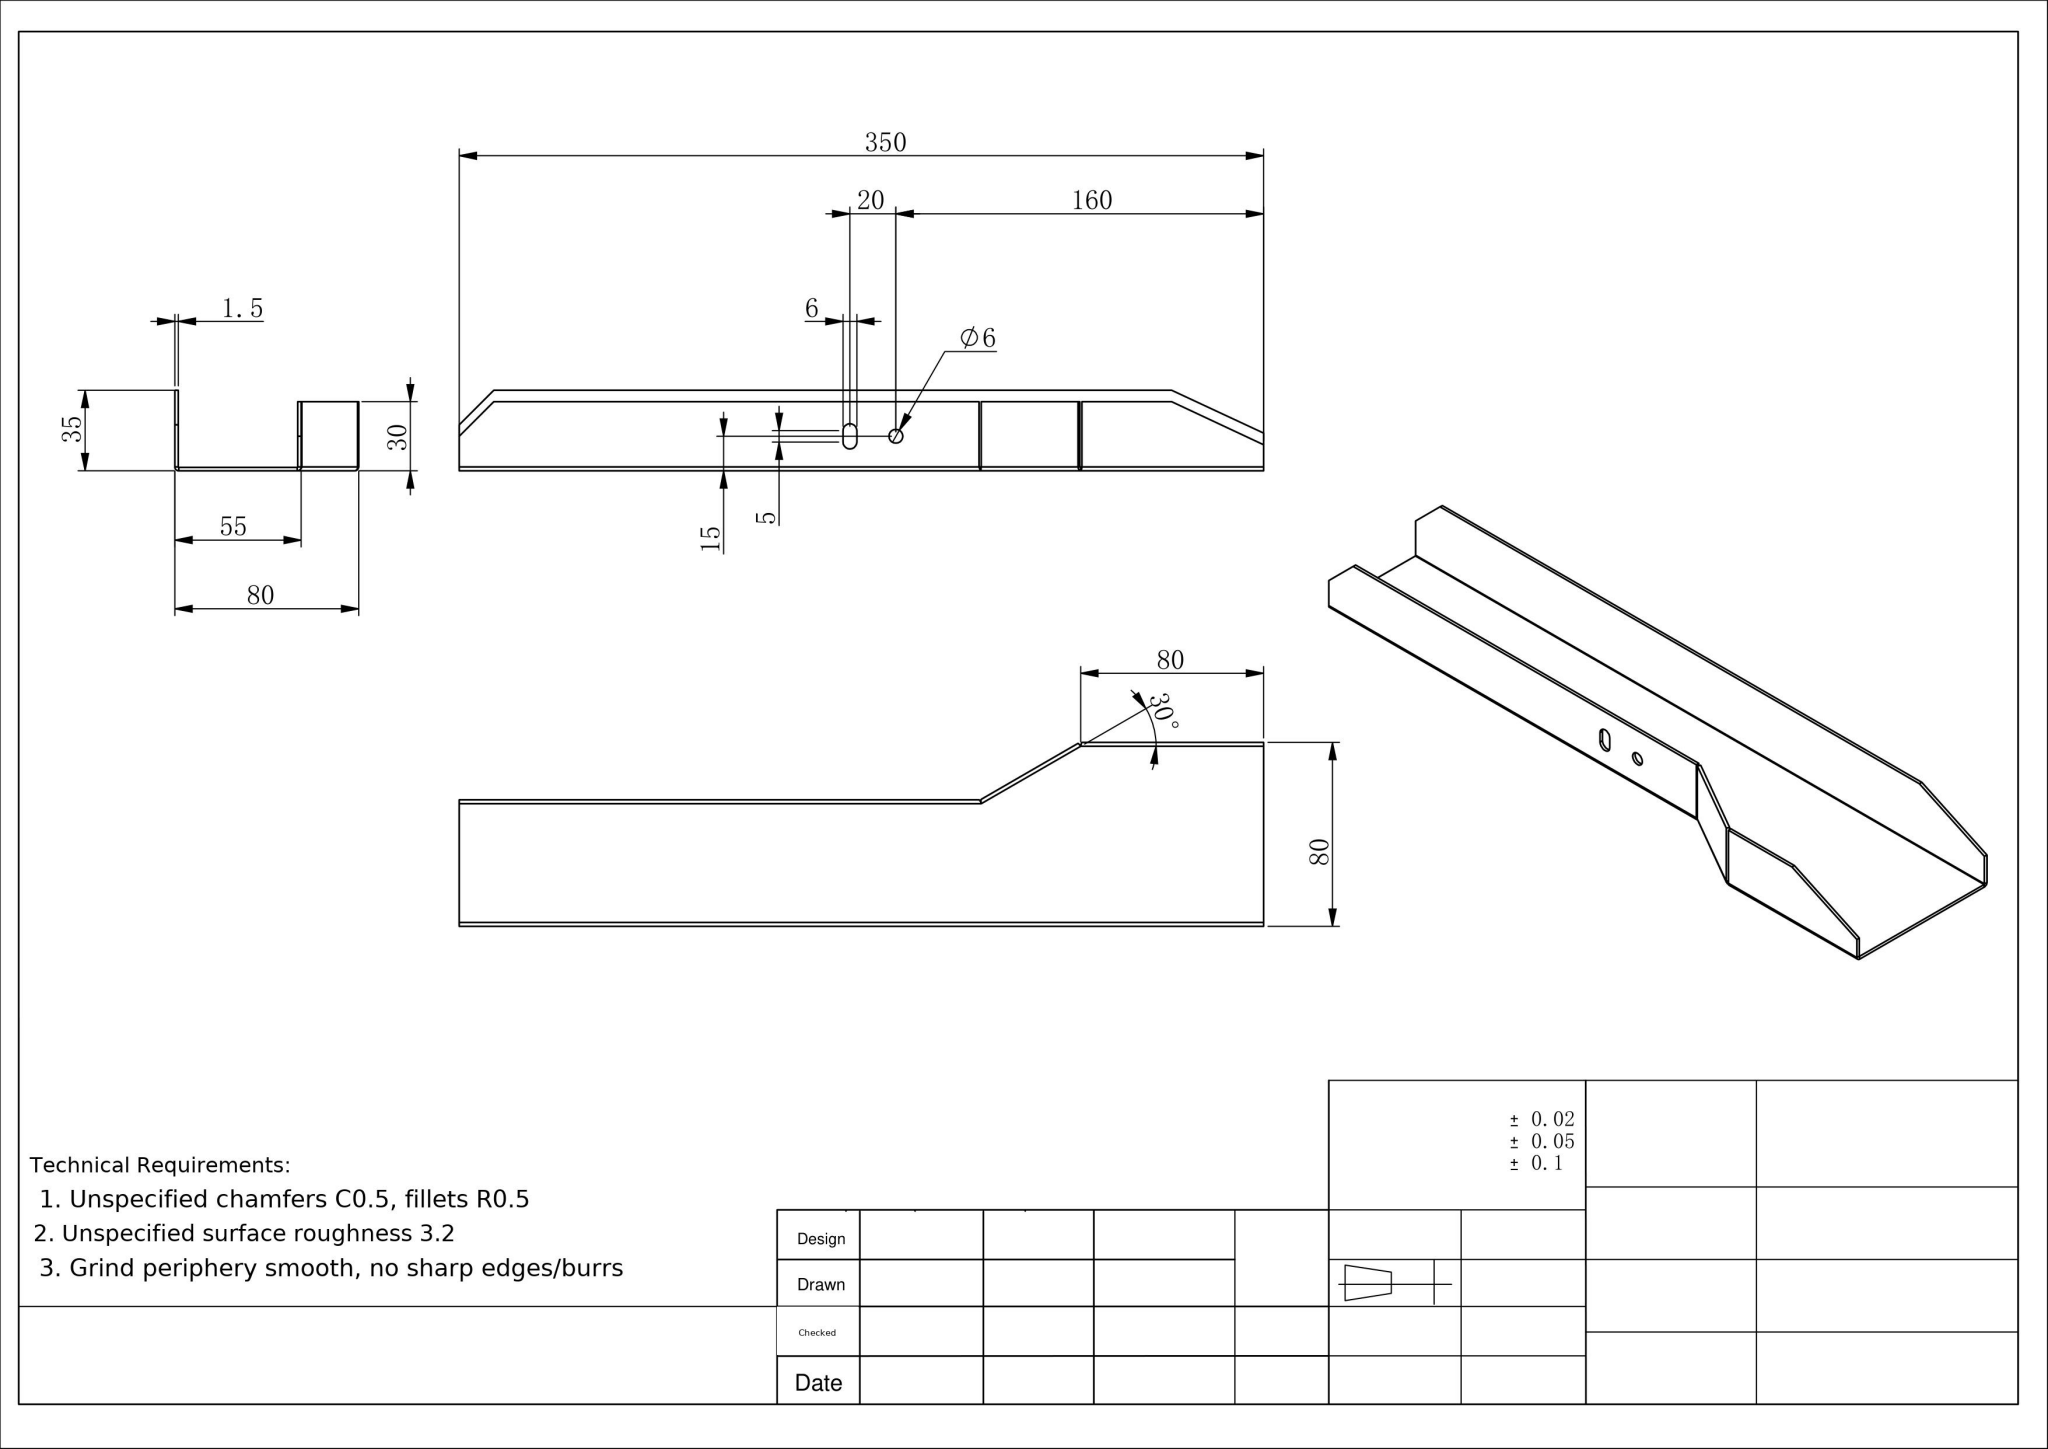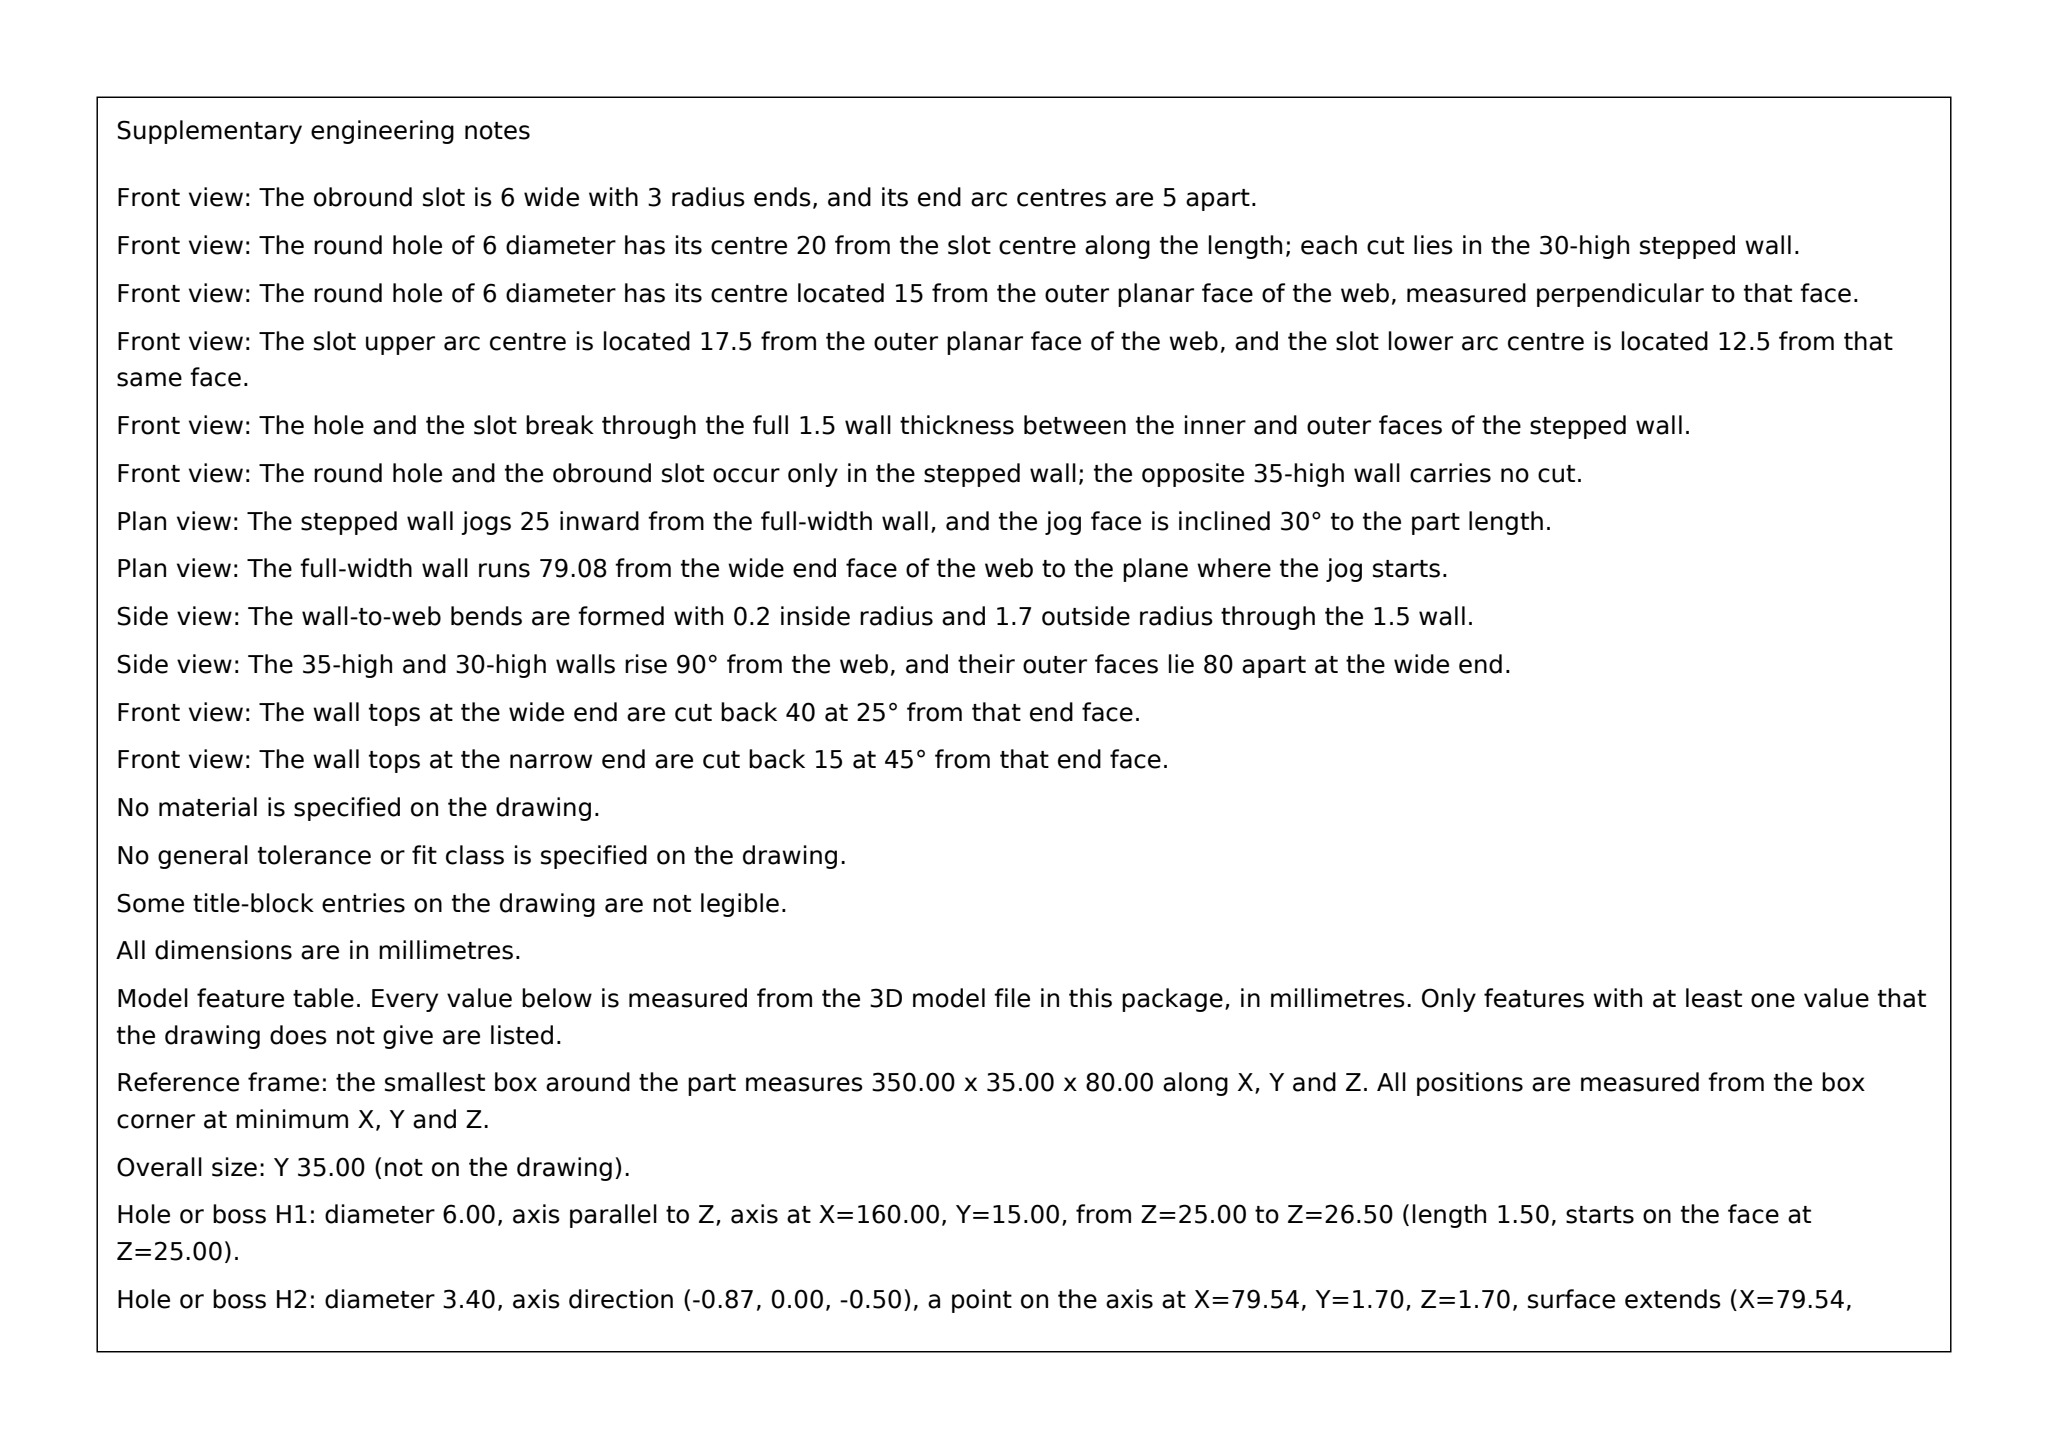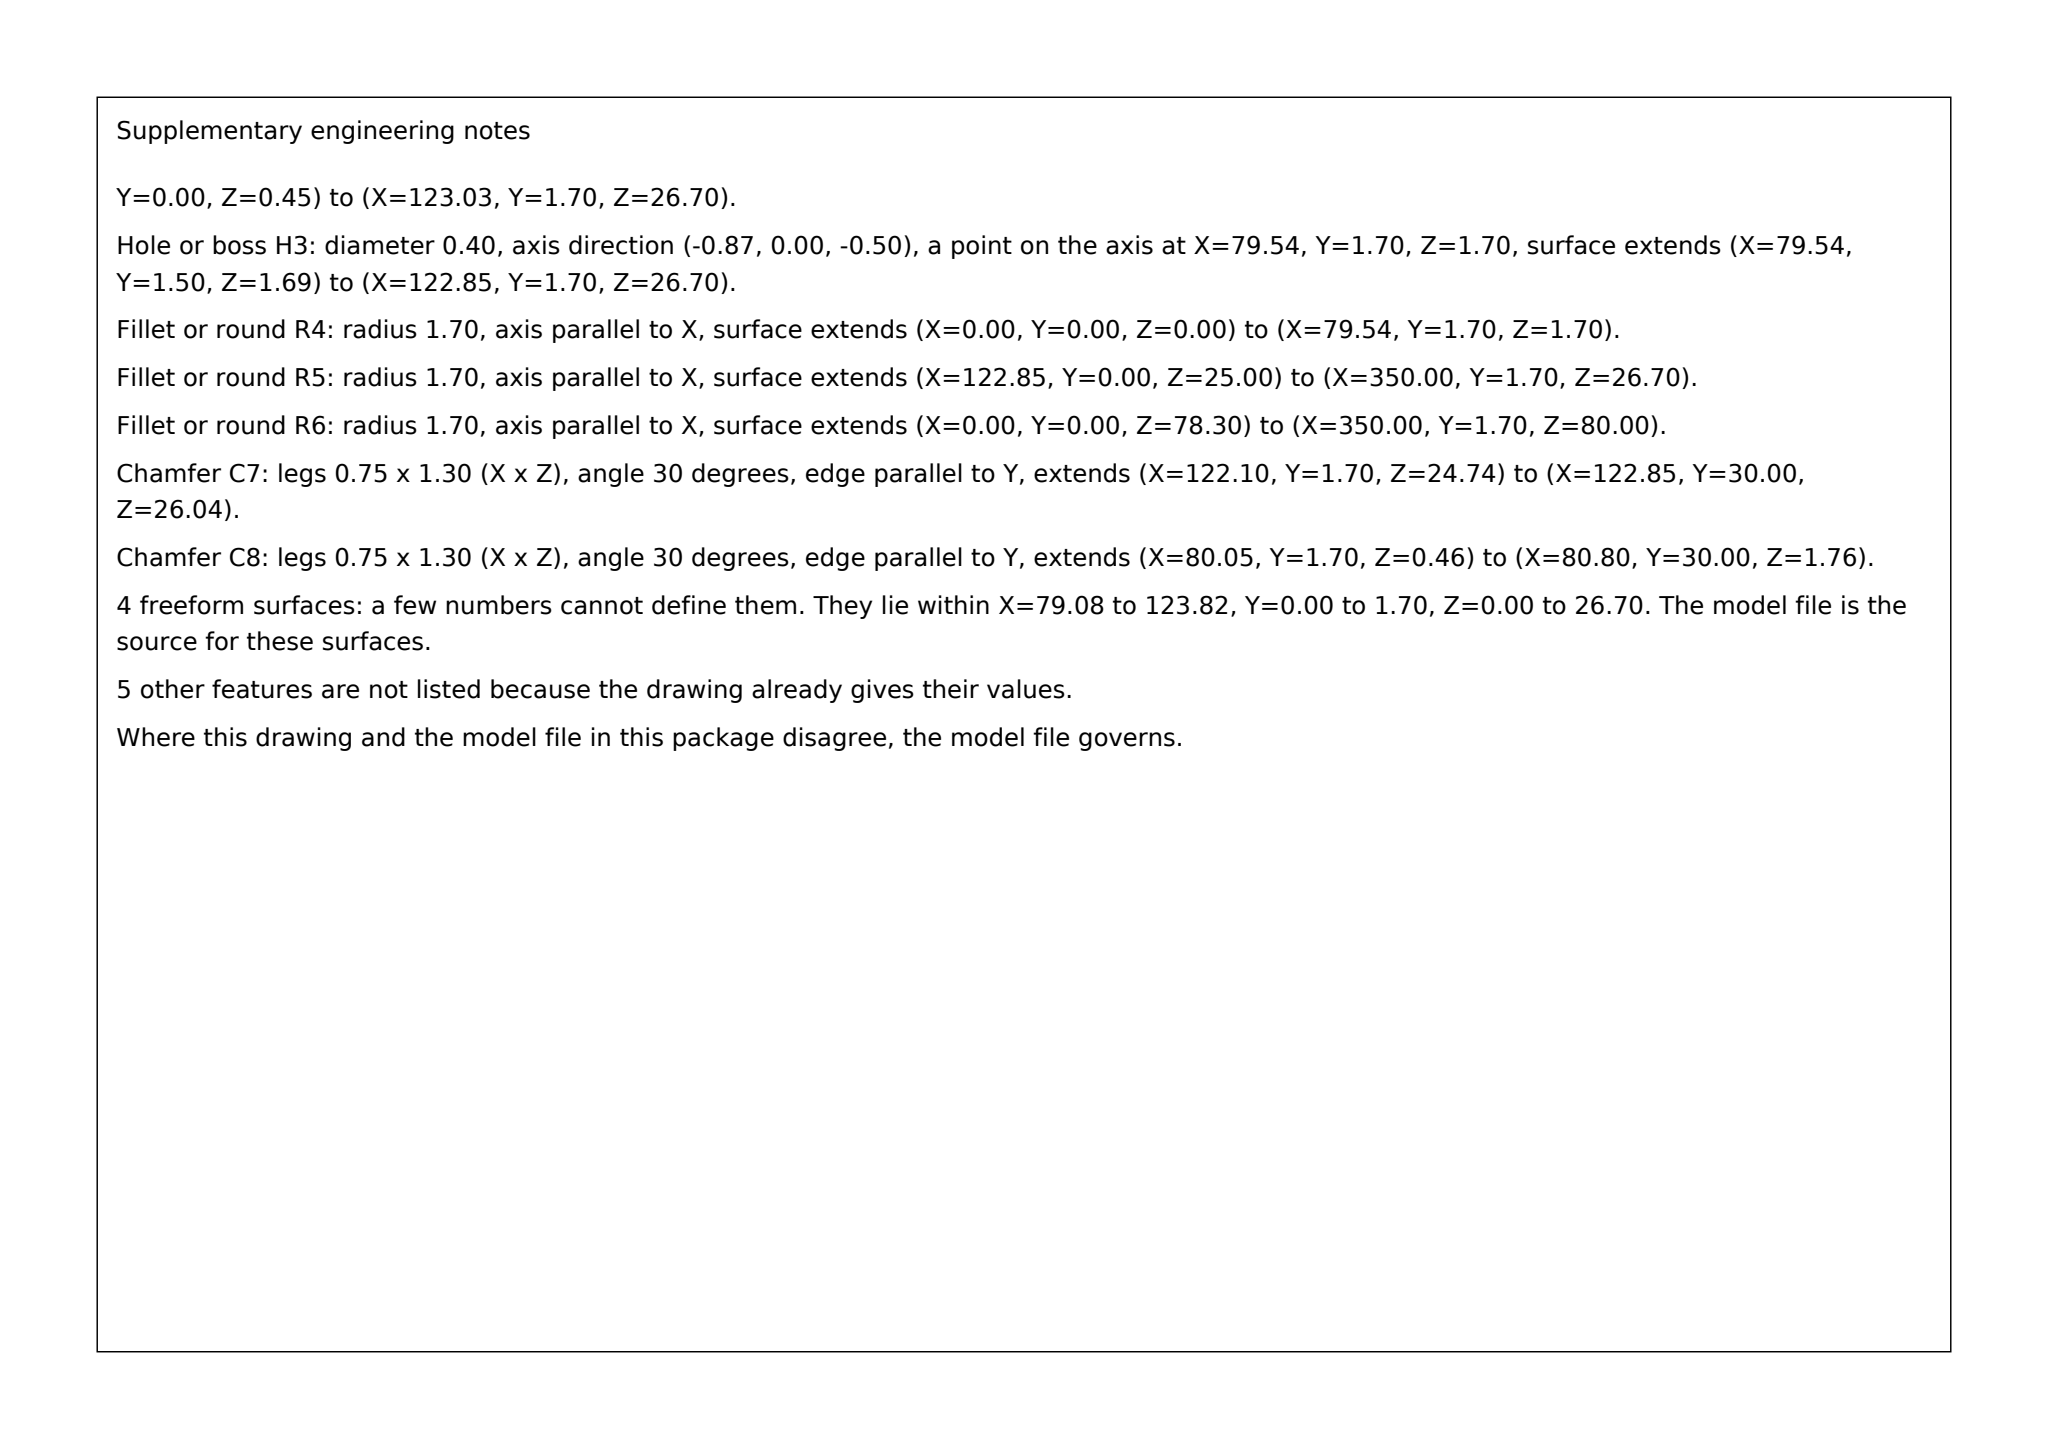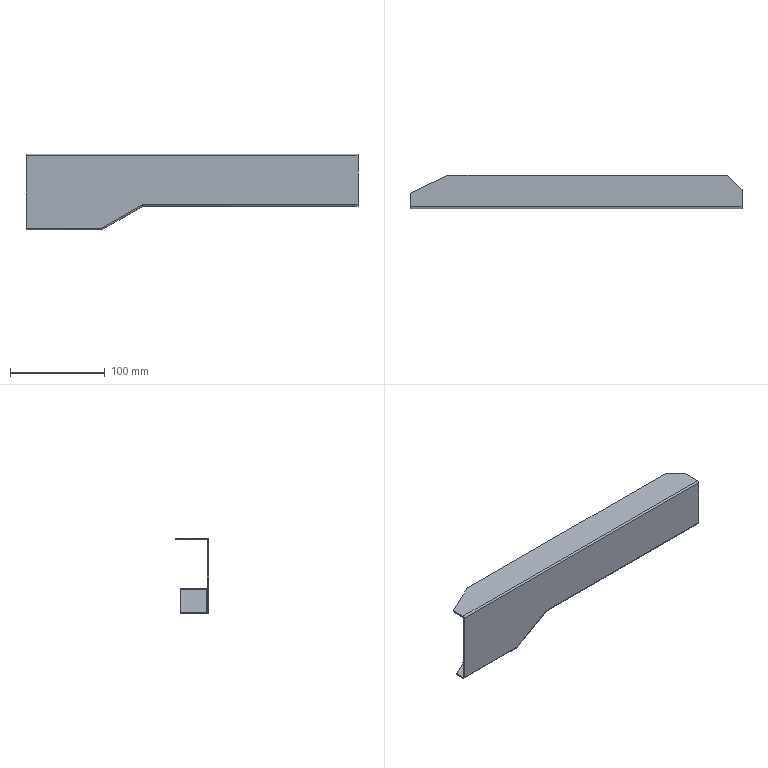Part | SolidWorks | mm | 1 solid | 51 faces | box 350 x 35 x 80 mm | volume 63379 mm3 | plane 34 | cylinder 13 | spline 4 | commonest cylinder face diameters 6 x5 0.4 x4 3.4 x4
Drawing notes:
ALL BEND RADII R1.7 INSIDE, R0.2 OUTSIDE (TYP ALL FOLDS) | from the solid: Cylinders dia 3.4 (R1.7) and dia 0.4 (R0.2) on x-axis at each fold line, e.g. [3.4,x,(1.72,1.72)] and [0.4,x,(1.72,26.72)]
ALL DIMS IN MM UNLESS OTHERWISE SPECIFIED | from the solid: STEP bbox 350.0 x 35.015 x 80.015 mm matches drawing values 350/35/80
LH END: CHAMFER 15 x 45° ON BOTH RAIL ENDS, 2 PL | from the solid: Front view is mirrored to STEP X (Ø6 hole at X=160, slot at X=180 from RH end). LH end = plane X=350 (5 faces); rail walls 1.5 thk at Z=0-1.5/25-26.5 and Z=78.5-80; top edge cut 15 run at 45° from X=350 inward.
RH END: CHAMFER 40 x 25° ON BOTH RAIL ENDS, 2 PL | from the solid: RH end = plane X=0 (5 faces), same end as Ø6 hole at X=160; sloped cut extends approx 40 in X from X=0 across both 1.5 thk rails (Z=0-1.5/25-26.5 and Z=78.5-80), 25° callout.